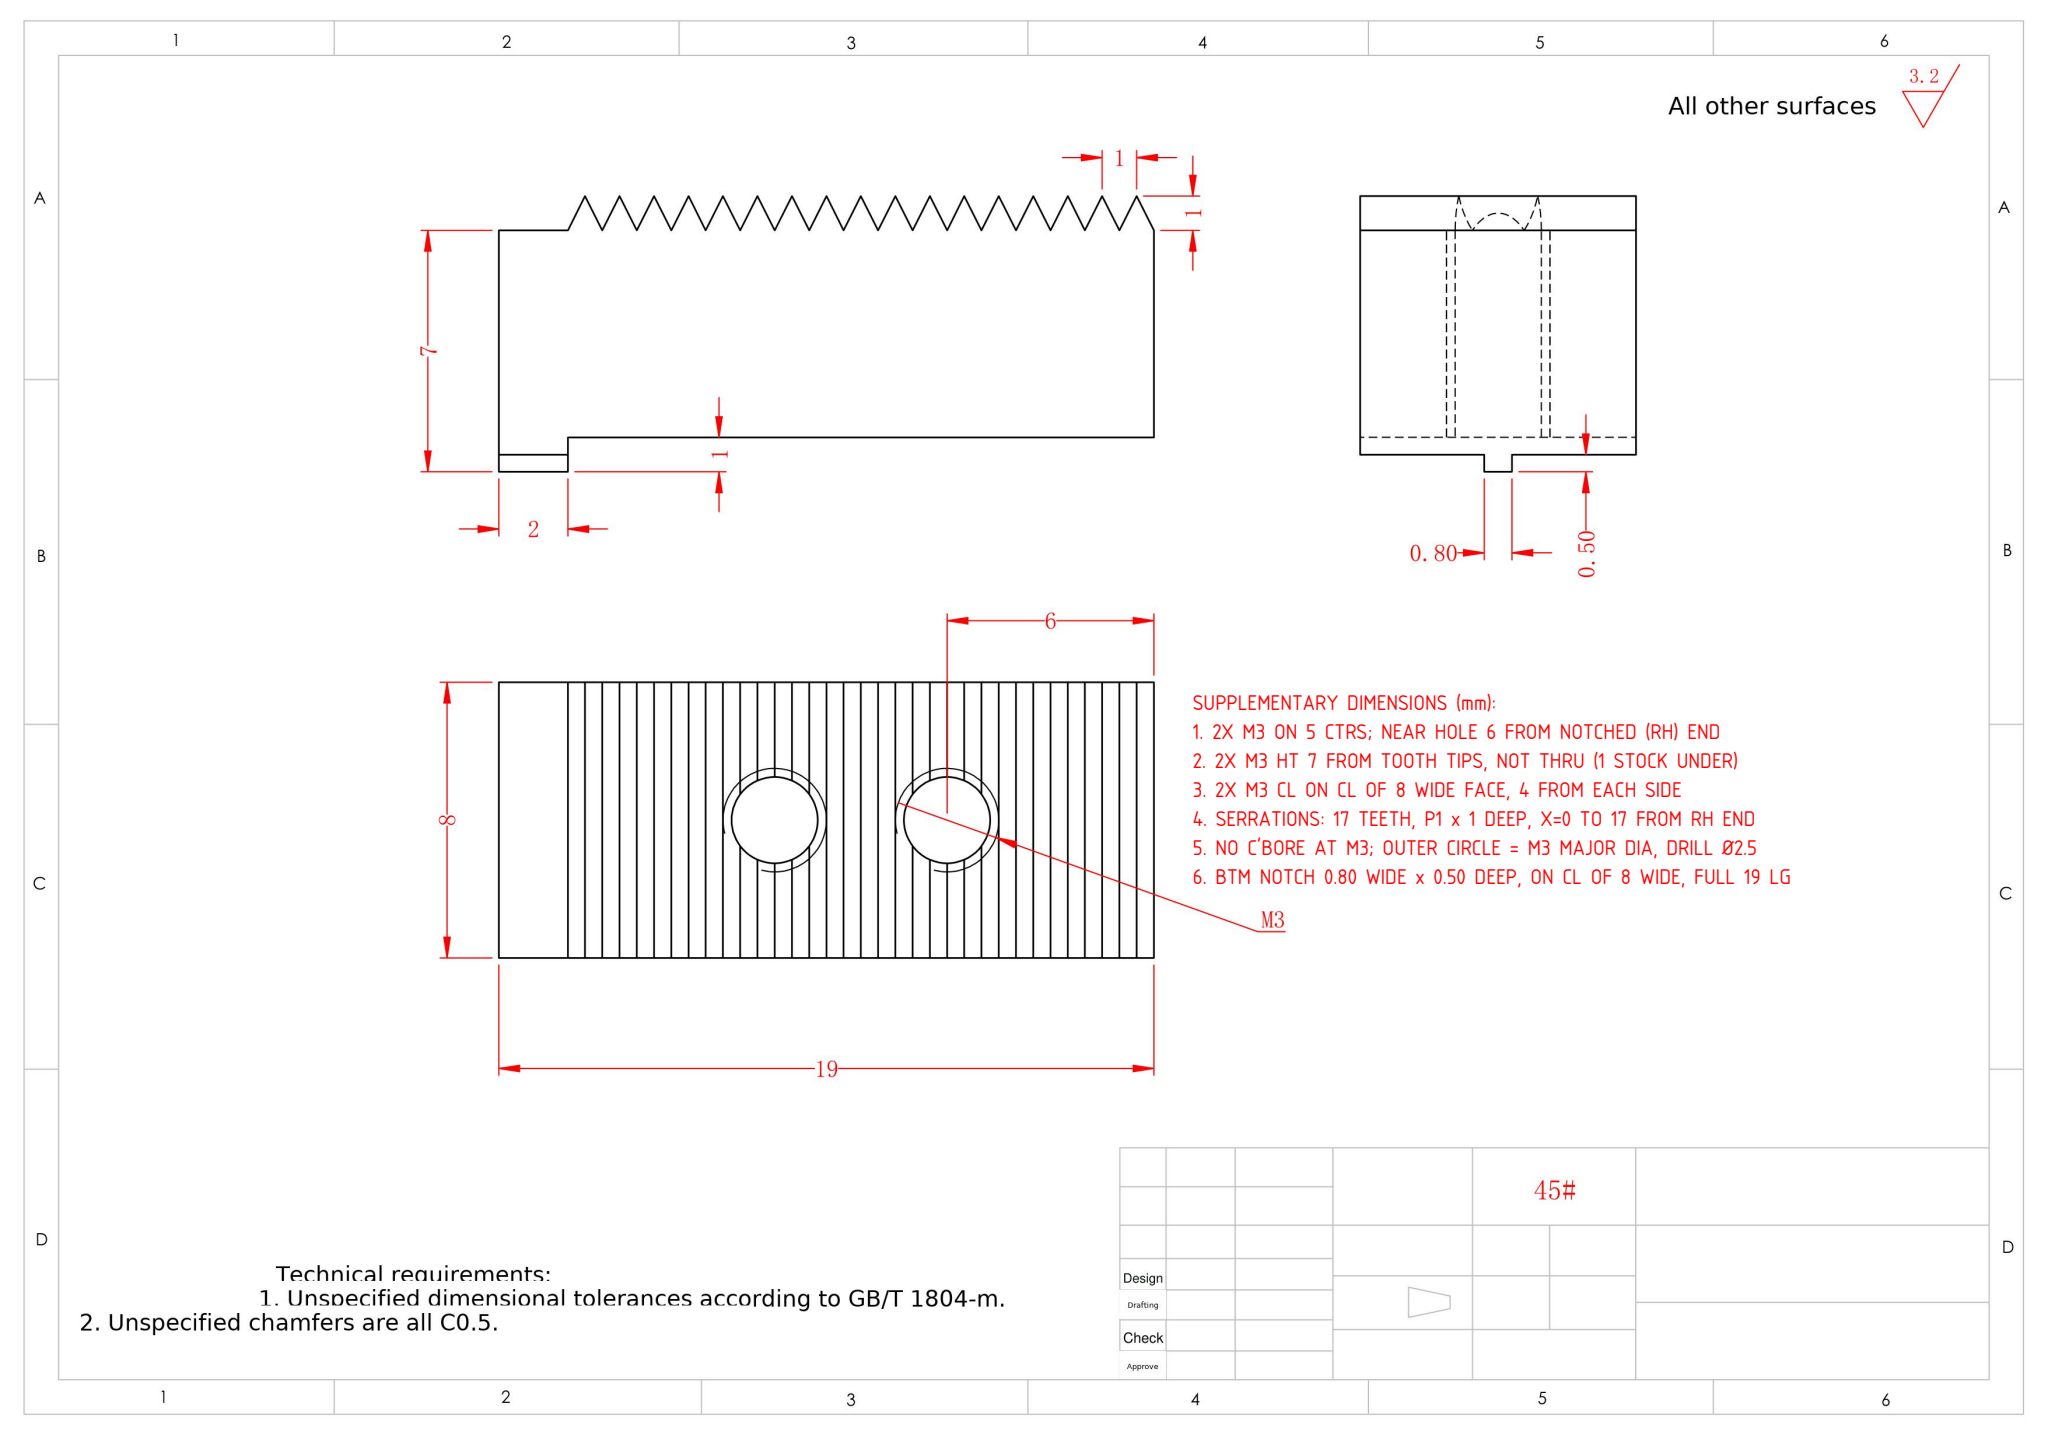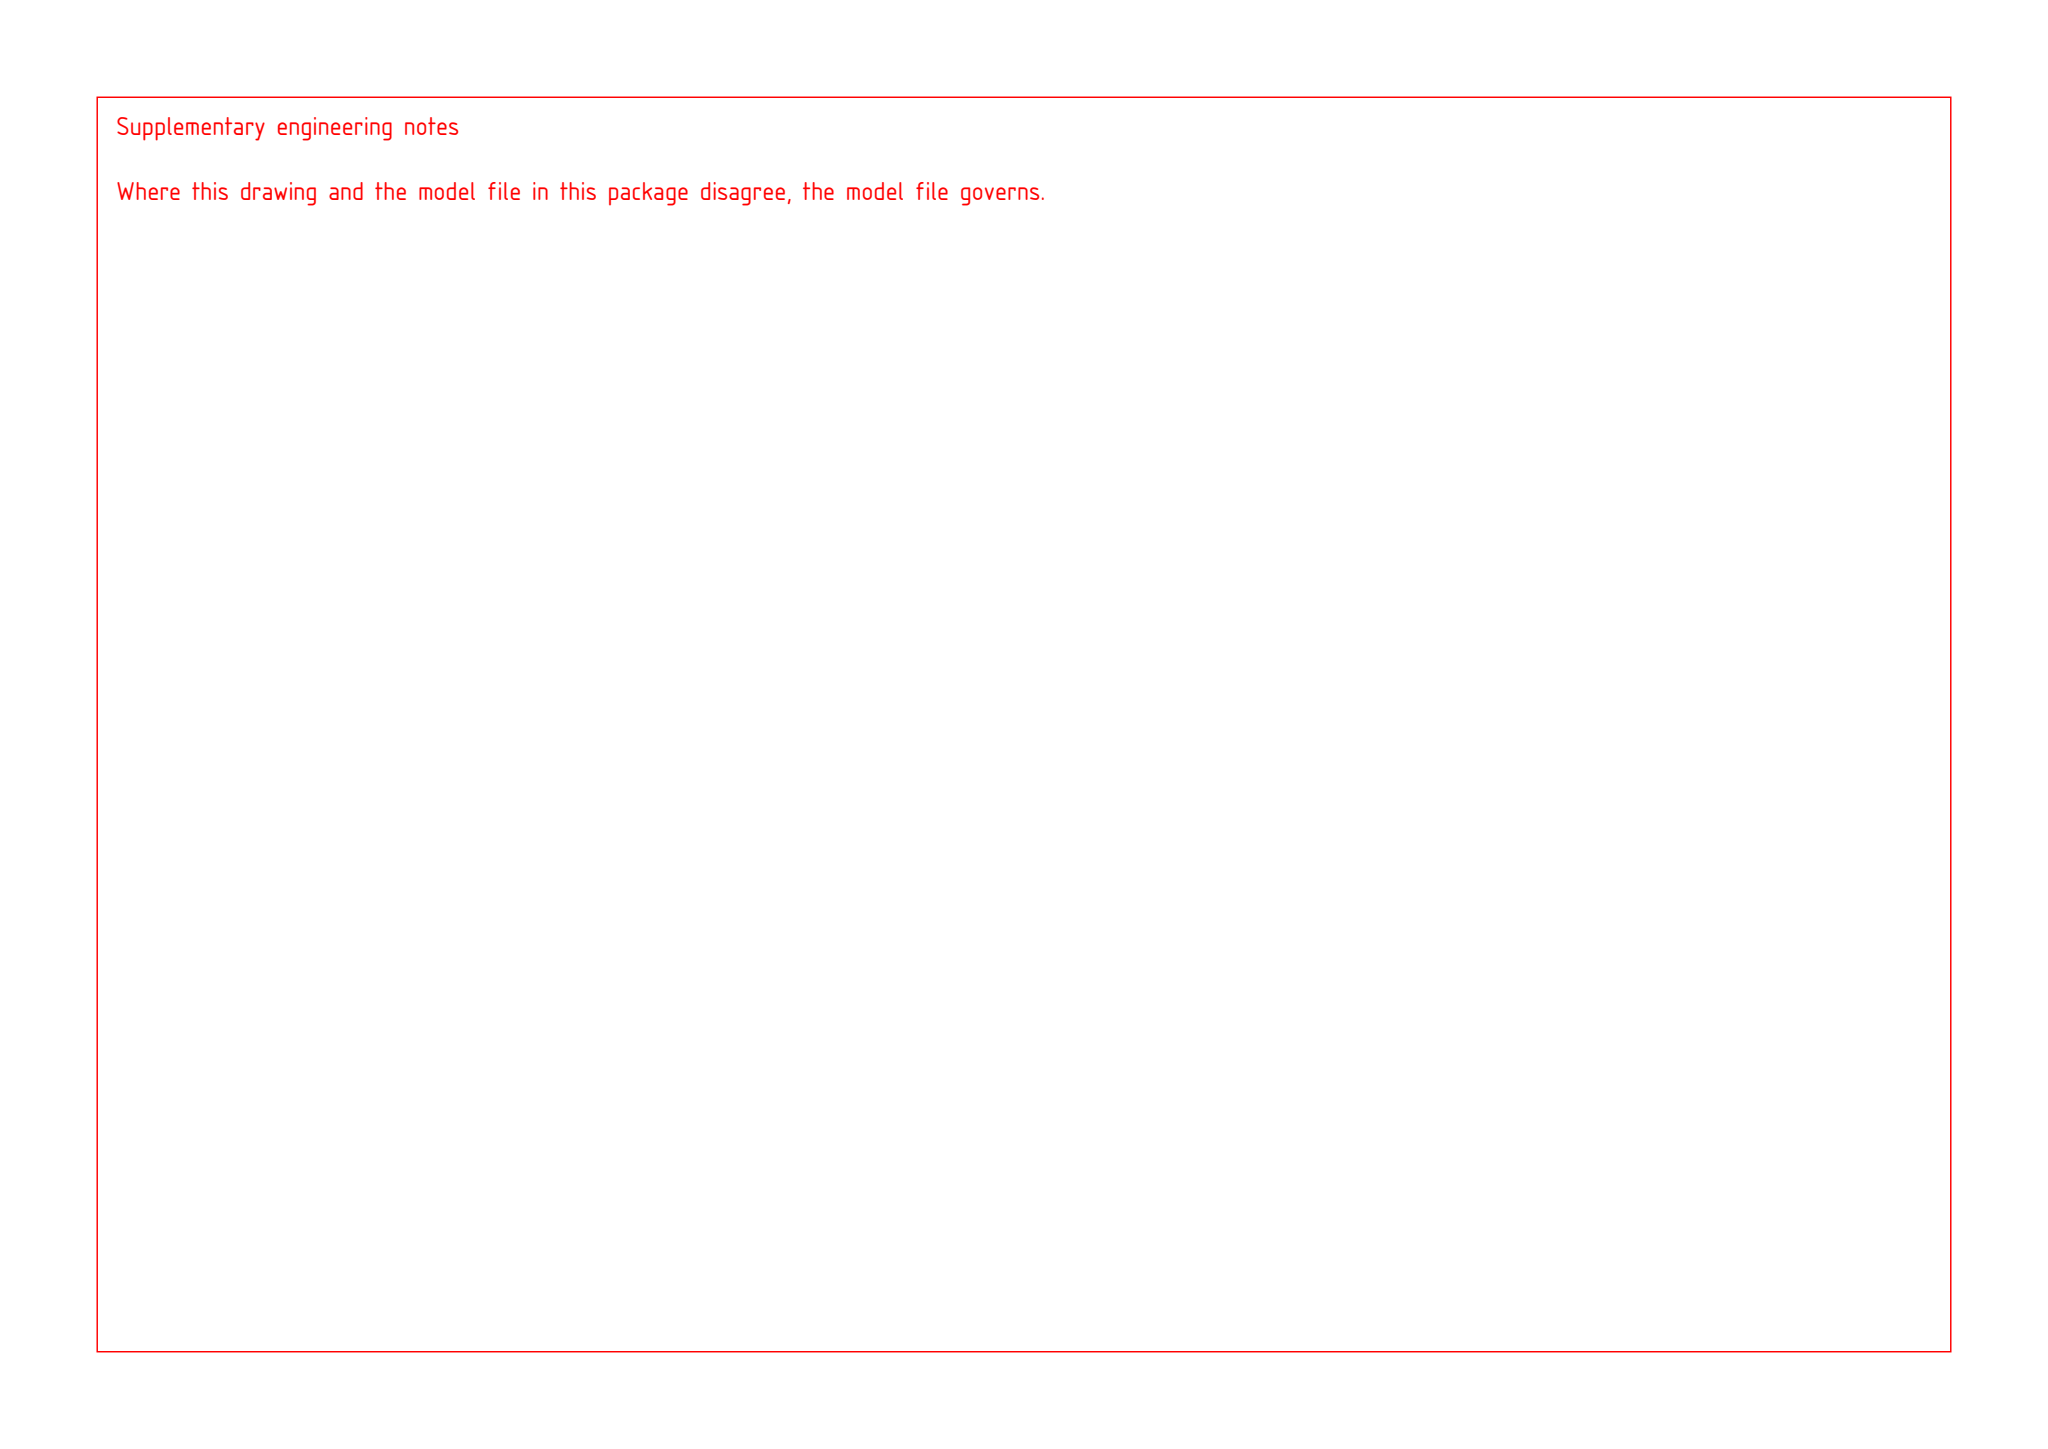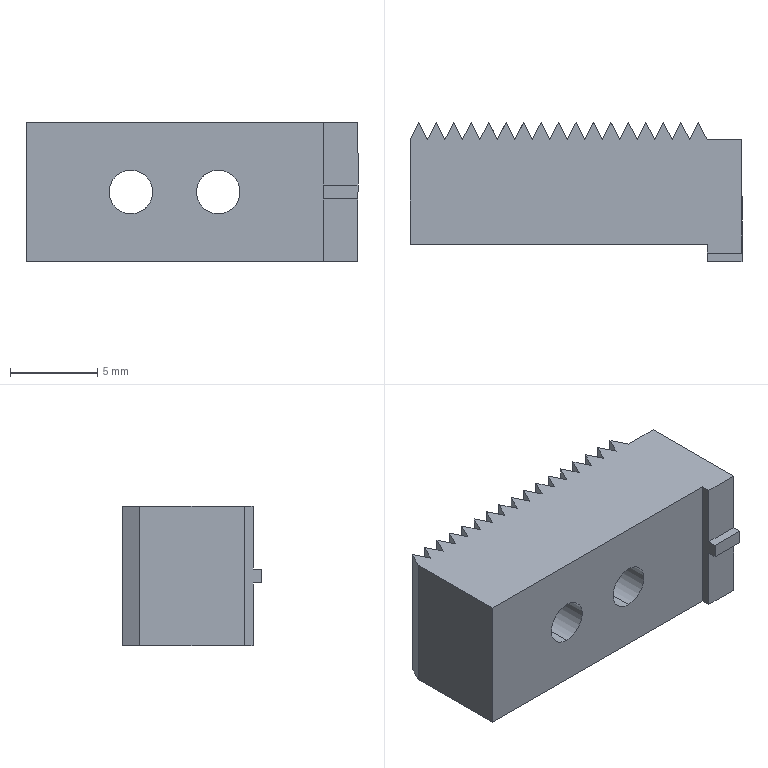Part | SolidWorks | mm | 1 solid | 58 faces | box 19 x 8 x 8 mm | volume 925 mm3 | plane 54 | cylinder 4 | commonest cylinder face diameters 2.5 x4
build123d program:
from build123d import *

# Parameters (mm, degrees)
BOSS_EXTRUDE1_DEPTH = 8
SKETCH2_W           = 10.567
SKETCH2_H           = 5.336
SKETCH2_W_2         = 6.915
SKETCH2_H_2         = 4.61
CUT_EXTRUDE1_DEPTH  = 0.5
BOSS_EXTRUDE3_DEPTH = 8
LPATTERN1_COUNT     = 17
LPATTERN1_PITCH     = 1
M3_TAPPED_HOLE1_D   = 2.5


with BuildPart() as part:
    # Sketch1 → Boss-Extrude1 (new body)
    with BuildSketch(Plane.XY):
        Polygon((0, 0), (19, 0), (19, -7), (17, -7), (17, -6), (0, -6), align=None)
    extrude(amount=BOSS_EXTRUDE1_DEPTH)

    # Sketch2 → Cut-Extrude1 (cut)
    with BuildSketch(Plane.XZ.offset(7)):
        with Locations((18.361, 7.068)):
            Rectangle(SKETCH2_W, SKETCH2_H)
        with Locations((15.588, 1.295)):
            Rectangle(SKETCH2_W_2, SKETCH2_H_2)
    extrude(amount=-CUT_EXTRUDE1_DEPTH, mode=Mode.SUBTRACT)

    # Sketch3 → Boss-Extrude3 (add)
    with BuildSketch(Plane.XY.offset(8)):
        Polygon((0, 0), (0.5, 1), (1, 0), align=None)
    boss_extrude3 = extrude(amount=-BOSS_EXTRUDE3_DEPTH)

    # LPattern1: Boss-Extrude3 ×17
    with Locations(*[(i * LPATTERN1_PITCH, 0, 0) for i in range(1, LPATTERN1_COUNT)]):
        add(boss_extrude3)

    # M3 Tapped Hole1 (through all)
    with Locations(Plane(origin=(0, -6, 0), x_dir=(-1, 0, 0), z_dir=(0, -1, 0))):
        with Locations((-6, -4), (-11, -4)):
            Hole(M3_TAPPED_HOLE1_D / 2)


solid = part.part